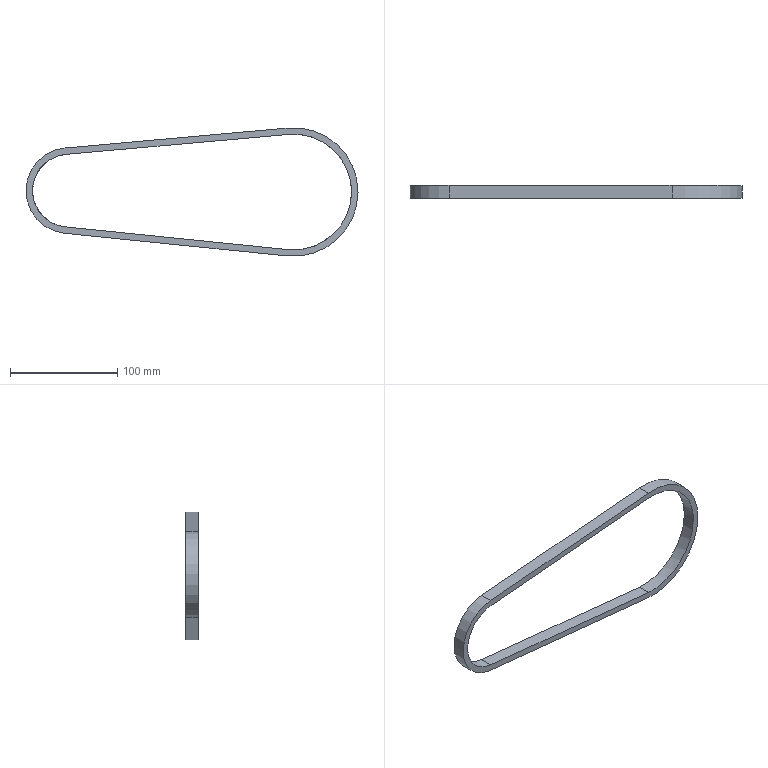Component | SolidWorks | LX-TSJ-09-1 | 1 solid | 12 faces | box 310 x 12 x 120 mm | volume 51639 mm3 | cylinder 6 | plane 6 | commonest cylinder face diameters 108 x2 120 x2 80 x1 68 x1
STEP:
#1=COLOUR_RGB('',0.7922,0.8196,0.9333);
#2=FILL_AREA_STYLE_COLOUR('',#1);
#3=FILL_AREA_STYLE('',(#2));
#4=SURFACE_STYLE_FILL_AREA(#3);
#5=SURFACE_SIDE_STYLE('',(#4));
#6=SURFACE_STYLE_USAGE(.BOTH.,#5);
#7=PRESENTATION_STYLE_ASSIGNMENT((#6));
#8=CARTESIAN_POINT('',(-5.033,-18.81,-14.193));
#9=VERTEX_POINT('',#8);
#10=CARTESIAN_POINT('',(-2.717,-18.81,-16.324));
#11=VERTEX_POINT('',#10);
#12=CARTESIAN_POINT('',(-4.843,-18.81,-16.311));
#13=DIRECTION('',(-0.,1.,0.));
#14=DIRECTION('',(-1.,0.,0.006108));
#15=AXIS2_PLACEMENT_3D('',#12,#13,#14);
#16=CIRCLE('',#15,2.126);
#17=EDGE_CURVE('',#9,#11,#16,.T.);
#18=ORIENTED_EDGE('',*,*,#17,.T.);
#19=CARTESIAN_POINT('',(-2.717,-19.282,-16.324));
#20=VERTEX_POINT('',#19);
#21=CARTESIAN_POINT('',(-2.717,-18.81,-16.324));
#22=DIRECTION('',(0.,-1.,-0.));
#23=VECTOR('',#22,39.37);
#24=LINE('',#21,#23);
#25=EDGE_CURVE('',#11,#20,#24,.T.);
#26=ORIENTED_EDGE('',*,*,#25,.T.);
#27=CARTESIAN_POINT('',(-5.033,-19.282,-14.193));
#28=VERTEX_POINT('',#27);
#29=CARTESIAN_POINT('',(-5.033,-19.282,-14.193));
#30=CARTESIAN_POINT('',(-4.885,-19.282,-14.18));
#31=CARTESIAN_POINT('',(-4.738,-19.282,-14.182));
#32=CARTESIAN_POINT('',(-4.444,-19.282,-14.218));
#33=CARTESIAN_POINT('',(-4.3,-19.282,-14.25));
#34=CARTESIAN_POINT('',(-4.02,-19.282,-14.345));
#35=CARTESIAN_POINT('',(-3.886,-19.282,-14.407));
#36=CARTESIAN_POINT('',(-3.631,-19.282,-14.558));
#37=CARTESIAN_POINT('',(-3.513,-19.282,-14.646));
#38=CARTESIAN_POINT('',(-3.295,-19.282,-14.847));
#39=CARTESIAN_POINT('',(-3.197,-19.282,-14.957));
#40=CARTESIAN_POINT('',(-3.026,-19.282,-15.199));
#41=CARTESIAN_POINT('',(-2.953,-19.282,-15.327));
#42=CARTESIAN_POINT('',(-2.835,-19.282,-15.598));
#43=CARTESIAN_POINT('',(-2.79,-19.282,-15.739));
#44=CARTESIAN_POINT('',(-2.731,-19.282,-16.029));
#45=CARTESIAN_POINT('',(-2.717,-19.282,-16.176));
#46=CARTESIAN_POINT('',(-2.717,-19.282,-16.324));
#47=B_SPLINE_CURVE_WITH_KNOTS('',3,(#29,#30,#31,#32,#33,#34,#35,#36,#37,#38,#39,#40,#41,#42,#43,#44,#45,#46),.UNSPECIFIED.,.F.,.F.,(4,2,2,2,2,2,2,2,4),(0.,0.0625,0.125,0.1875,0.25,0.3125,0.375,0.4375,0.5),.UNSPECIFIED.);
#48=EDGE_CURVE('',#28,#20,#47,.T.);
#49=ORIENTED_EDGE('',*,*,#48,.F.);
#50=CARTESIAN_POINT('',(-5.033,-18.81,-14.193));
#51=DIRECTION('',(0.,-1.,-0.));
#52=VECTOR('',#51,39.37);
#53=LINE('',#50,#52);
#54=EDGE_CURVE('',#9,#28,#53,.T.);
#55=ORIENTED_EDGE('',*,*,#54,.F.);
#56=EDGE_LOOP('',(#18,#26,#49,#55));
#57=FACE_OUTER_BOUND('',#56,.T.);
#58=CARTESIAN_POINT('',(-4.843,-18.81,-16.311));
#59=DIRECTION('',(0.,-1.,-0.));
#60=DIRECTION('',(1.,0.,-0.006108));
#61=AXIS2_PLACEMENT_3D('',#58,#59,#60);
#62=CYLINDRICAL_SURFACE('',#61,2.126);
#63=ADVANCED_FACE('',(#57),#62,.F.);
#64=CARTESIAN_POINT('',(-5.083,-18.81,-18.661));
#65=VERTEX_POINT('',#64);
#66=CARTESIAN_POINT('',(-2.481,-18.81,-16.325));
#67=VERTEX_POINT('',#66);
#68=CARTESIAN_POINT('',(-4.843,-18.81,-16.311));
#69=DIRECTION('',(0.,-1.,-0.));
#70=DIRECTION('',(1.,0.,-0.006108));
#71=AXIS2_PLACEMENT_3D('',#68,#69,#70);
#72=CIRCLE('',#71,2.362);
#73=EDGE_CURVE('',#65,#67,#72,.T.);
#74=ORIENTED_EDGE('',*,*,#73,.T.);
#75=CARTESIAN_POINT('',(-2.481,-19.282,-16.325));
#76=VERTEX_POINT('',#75);
#77=CARTESIAN_POINT('',(-2.481,-18.81,-16.325));
#78=DIRECTION('',(0.,-1.,-0.));
#79=VECTOR('',#78,39.37);
#80=LINE('',#77,#79);
#81=EDGE_CURVE('',#67,#76,#80,.T.);
#82=ORIENTED_EDGE('',*,*,#81,.T.);
#83=CARTESIAN_POINT('',(-5.083,-19.282,-18.661));
#84=VERTEX_POINT('',#83);
#85=CARTESIAN_POINT('',(-4.843,-19.282,-16.311));
#86=DIRECTION('',(-0.,1.,0.));
#87=DIRECTION('',(1.,0.,-0.006108));
#88=AXIS2_PLACEMENT_3D('',#85,#86,#87);
#89=CIRCLE('',#88,2.362);
#90=EDGE_CURVE('',#76,#84,#89,.T.);
#91=ORIENTED_EDGE('',*,*,#90,.T.);
#92=CARTESIAN_POINT('',(-5.083,-18.81,-18.661));
#93=DIRECTION('',(0.,-1.,-0.));
#94=VECTOR('',#93,39.37);
#95=LINE('',#92,#94);
#96=EDGE_CURVE('',#65,#84,#95,.T.);
#97=ORIENTED_EDGE('',*,*,#96,.F.);
#98=EDGE_LOOP('',(#74,#82,#91,#97));
#99=FACE_OUTER_BOUND('',#98,.T.);
#100=CARTESIAN_POINT('',(-4.843,-18.81,-16.311));
#101=DIRECTION('',(0.,-1.,-0.));
#102=DIRECTION('',(1.,0.,-0.006108));
#103=AXIS2_PLACEMENT_3D('',#100,#101,#102);
#104=CYLINDRICAL_SURFACE('',#103,2.362);
#105=ADVANCED_FACE('',(#99),#104,.T.);
#106=CARTESIAN_POINT('',(-13.251,-18.81,-14.692));
#107=VERTEX_POINT('',#106);
#108=CARTESIAN_POINT('',(-5.054,-18.81,-13.958));
#109=VERTEX_POINT('',#108);
#110=CARTESIAN_POINT('',(-13.251,-18.81,-14.692));
#111=DIRECTION('',(0.996,-0.,0.08916));
#112=VECTOR('',#111,39.37);
#113=LINE('',#110,#112);
#114=EDGE_CURVE('',#107,#109,#113,.T.);
#115=ORIENTED_EDGE('',*,*,#114,.T.);
#116=CARTESIAN_POINT('',(-4.843,-18.81,-16.311));
#117=DIRECTION('',(0.,-1.,-0.));
#118=DIRECTION('',(1.,0.,-0.006108));
#119=AXIS2_PLACEMENT_3D('',#116,#117,#118);
#120=CIRCLE('',#119,2.362);
#121=EDGE_CURVE('',#67,#109,#120,.T.);
#122=ORIENTED_EDGE('',*,*,#121,.F.);
#123=ORIENTED_EDGE('',*,*,#73,.F.);
#124=CARTESIAN_POINT('',(-13.271,-18.81,-17.827));
#125=VERTEX_POINT('',#124);
#126=CARTESIAN_POINT('',(-5.083,-18.81,-18.661));
#127=DIRECTION('',(-0.9949,-0.,0.1013));
#128=VECTOR('',#127,39.37);
#129=LINE('',#126,#128);
#130=EDGE_CURVE('',#65,#125,#129,.T.);
#131=ORIENTED_EDGE('',*,*,#130,.T.);
#132=CARTESIAN_POINT('',(-13.111,-18.81,-16.26));
#133=DIRECTION('',(-0.,1.,0.));
#134=DIRECTION('',(-1.,0.,0.006108));
#135=AXIS2_PLACEMENT_3D('',#132,#133,#134);
#136=CIRCLE('',#135,1.575);
#137=EDGE_CURVE('',#125,#107,#136,.T.);
#138=ORIENTED_EDGE('',*,*,#137,.T.);
#139=EDGE_LOOP('',(#115,#122,#123,#131,#138));
#140=FACE_OUTER_BOUND('',#139,.T.);
#141=CARTESIAN_POINT('',(-5.059,-18.81,-18.426));
#142=VERTEX_POINT('',#141);
#143=CARTESIAN_POINT('',(-13.247,-18.81,-17.592));
#144=VERTEX_POINT('',#143);
#145=CARTESIAN_POINT('',(-5.059,-18.81,-18.426));
#146=DIRECTION('',(-0.9949,-0.,0.1013));
#147=VECTOR('',#146,39.37);
#148=LINE('',#145,#147);
#149=EDGE_CURVE('',#142,#144,#148,.T.);
#150=ORIENTED_EDGE('',*,*,#149,.F.);
#151=CARTESIAN_POINT('',(-4.843,-18.81,-16.311));
#152=DIRECTION('',(-0.,1.,0.));
#153=DIRECTION('',(-1.,0.,0.006108));
#154=AXIS2_PLACEMENT_3D('',#151,#152,#153);
#155=CIRCLE('',#154,2.126);
#156=EDGE_CURVE('',#11,#142,#155,.T.);
#157=ORIENTED_EDGE('',*,*,#156,.F.);
#158=ORIENTED_EDGE('',*,*,#17,.F.);
#159=CARTESIAN_POINT('',(-13.23,-18.81,-14.927));
#160=VERTEX_POINT('',#159);
#161=CARTESIAN_POINT('',(-13.23,-18.81,-14.927));
#162=DIRECTION('',(0.996,-0.,0.08916));
#163=VECTOR('',#162,39.37);
#164=LINE('',#161,#163);
#165=EDGE_CURVE('',#160,#9,#164,.T.);
#166=ORIENTED_EDGE('',*,*,#165,.F.);
#167=CARTESIAN_POINT('',(-13.111,-18.81,-16.26));
#168=DIRECTION('',(-0.,1.,0.));
#169=DIRECTION('',(-1.,0.,0.006108));
#170=AXIS2_PLACEMENT_3D('',#167,#168,#169);
#171=CIRCLE('',#170,1.339);
#172=EDGE_CURVE('',#144,#160,#171,.T.);
#173=ORIENTED_EDGE('',*,*,#172,.F.);
#174=EDGE_LOOP('',(#150,#157,#158,#166,#173));
#175=FACE_BOUND('',#174,.T.);
#176=CARTESIAN_POINT('',(-4.843,-18.81,-16.311));
#177=DIRECTION('',(-0.,1.,0.));
#178=DIRECTION('',(-1.,-0.,0.006108));
#179=AXIS2_PLACEMENT_3D('',#176,#177,#178);
#180=PLANE('',#179);
#181=ADVANCED_FACE('',(#140,#175),#180,.T.);
#182=CARTESIAN_POINT('',(-13.23,-19.282,-14.927));
#183=VERTEX_POINT('',#182);
#184=CARTESIAN_POINT('',(-13.23,-19.282,-14.927));
#185=DIRECTION('',(0.996,-0.,0.08916));
#186=VECTOR('',#185,39.37);
#187=LINE('',#184,#186);
#188=EDGE_CURVE('',#183,#28,#187,.T.);
#189=ORIENTED_EDGE('',*,*,#188,.T.);
#190=ORIENTED_EDGE('',*,*,#48,.T.);
#191=CARTESIAN_POINT('',(-5.059,-19.282,-18.426));
#192=VERTEX_POINT('',#191);
#193=CARTESIAN_POINT('',(-2.717,-19.282,-16.324));
#194=CARTESIAN_POINT('',(-2.718,-19.282,-16.472));
#195=CARTESIAN_POINT('',(-2.735,-19.282,-16.619));
#196=CARTESIAN_POINT('',(-2.798,-19.282,-16.908));
#197=CARTESIAN_POINT('',(-2.844,-19.282,-17.048));
#198=CARTESIAN_POINT('',(-2.965,-19.282,-17.318));
#199=CARTESIAN_POINT('',(-3.039,-19.282,-17.445));
#200=CARTESIAN_POINT('',(-3.214,-19.282,-17.685));
#201=CARTESIAN_POINT('',(-3.313,-19.282,-17.794));
#202=CARTESIAN_POINT('',(-3.533,-19.282,-17.992));
#203=CARTESIAN_POINT('',(-3.653,-19.282,-18.078));
#204=CARTESIAN_POINT('',(-3.909,-19.282,-18.226));
#205=CARTESIAN_POINT('',(-4.044,-19.282,-18.286));
#206=CARTESIAN_POINT('',(-4.325,-19.282,-18.378));
#207=CARTESIAN_POINT('',(-4.47,-19.282,-18.409));
#208=CARTESIAN_POINT('',(-4.764,-19.282,-18.441));
#209=CARTESIAN_POINT('',(-4.911,-19.282,-18.441));
#210=CARTESIAN_POINT('',(-5.059,-19.282,-18.426));
#211=B_SPLINE_CURVE_WITH_KNOTS('',3,(#193,#194,#195,#196,#197,#198,#199,#200,#201,#202,#203,#204,#205,#206,#207,#208,#209,#210),.UNSPECIFIED.,.F.,.F.,(4,2,2,2,2,2,2,2,4),(0.5,0.5625,0.625,0.6875,0.75,0.8125,0.875,0.9375,1.),.UNSPECIFIED.);
#212=EDGE_CURVE('',#20,#192,#211,.T.);
#213=ORIENTED_EDGE('',*,*,#212,.T.);
#214=CARTESIAN_POINT('',(-13.247,-19.282,-17.592));
#215=VERTEX_POINT('',#214);
#216=CARTESIAN_POINT('',(-5.059,-19.282,-18.426));
#217=DIRECTION('',(-0.9949,-0.,0.1013));
#218=VECTOR('',#217,39.37);
#219=LINE('',#216,#218);
#220=EDGE_CURVE('',#192,#215,#219,.T.);
#221=ORIENTED_EDGE('',*,*,#220,.T.);
#222=CARTESIAN_POINT('',(-13.247,-19.282,-17.592));
#223=CARTESIAN_POINT('',(-13.329,-19.282,-17.584));
#224=CARTESIAN_POINT('',(-13.409,-19.282,-17.568));
#225=CARTESIAN_POINT('',(-13.568,-19.282,-17.521));
#226=CARTESIAN_POINT('',(-13.644,-19.282,-17.491));
#227=CARTESIAN_POINT('',(-13.791,-19.282,-17.416));
#228=CARTESIAN_POINT('',(-13.861,-19.282,-17.372));
#229=CARTESIAN_POINT('',(-13.992,-19.282,-17.272));
#230=CARTESIAN_POINT('',(-14.052,-19.282,-17.216));
#231=CARTESIAN_POINT('',(-14.162,-19.282,-17.093));
#232=CARTESIAN_POINT('',(-14.211,-19.282,-17.027));
#233=CARTESIAN_POINT('',(-14.297,-19.282,-16.886));
#234=CARTESIAN_POINT('',(-14.333,-19.282,-16.813));
#235=CARTESIAN_POINT('',(-14.392,-19.282,-16.658));
#236=CARTESIAN_POINT('',(-14.414,-19.282,-16.579));
#237=CARTESIAN_POINT('',(-14.443,-19.282,-16.417));
#238=CARTESIAN_POINT('',(-14.45,-19.282,-16.335));
#239=CARTESIAN_POINT('',(-14.449,-19.282,-16.17));
#240=CARTESIAN_POINT('',(-14.441,-19.282,-16.088));
#241=CARTESIAN_POINT('',(-14.41,-19.282,-15.926));
#242=CARTESIAN_POINT('',(-14.387,-19.282,-15.847));
#243=CARTESIAN_POINT('',(-14.326,-19.282,-15.693));
#244=CARTESIAN_POINT('',(-14.289,-19.282,-15.62));
#245=CARTESIAN_POINT('',(-14.202,-19.282,-15.48));
#246=CARTESIAN_POINT('',(-14.152,-19.282,-15.415));
#247=CARTESIAN_POINT('',(-14.04,-19.282,-15.293));
#248=CARTESIAN_POINT('',(-13.979,-19.282,-15.238));
#249=CARTESIAN_POINT('',(-13.847,-19.282,-15.139));
#250=CARTESIAN_POINT('',(-13.777,-19.282,-15.096));
#251=CARTESIAN_POINT('',(-13.629,-19.282,-15.023));
#252=CARTESIAN_POINT('',(-13.552,-19.282,-14.994));
#253=CARTESIAN_POINT('',(-13.393,-19.282,-14.949));
#254=CARTESIAN_POINT('',(-13.312,-19.282,-14.935));
#255=CARTESIAN_POINT('',(-13.23,-19.282,-14.927));
#256=B_SPLINE_CURVE_WITH_KNOTS('',3,(#222,#223,#224,#225,#226,#227,#228,#229,#230,#231,#232,#233,#234,#235,#236,#237,#238,#239,#240,#241,#242,#243,#244,#245,#246,#247,#248,#249,#250,#251,#252,#253,#254,#255),.UNSPECIFIED.,.F.,.F.,(4,2,2,2,2,2,2,2,2,2,2,2,2,2,2,2,4),(0.,0.0625,0.125,0.1875,0.25,0.3125,0.375,0.4375,0.5,0.5625,0.625,0.6875,0.75,0.8125,0.875,0.9375,1.),.UNSPECIFIED.);
#257=EDGE_CURVE('',#215,#183,#256,.T.);
#258=ORIENTED_EDGE('',*,*,#257,.T.);
#259=EDGE_LOOP('',(#189,#190,#213,#221,#258));
#260=FACE_BOUND('',#259,.T.);
#261=CARTESIAN_POINT('',(-5.054,-19.282,-13.958));
#262=VERTEX_POINT('',#261);
#263=CARTESIAN_POINT('',(-4.843,-19.282,-16.311));
#264=DIRECTION('',(-0.,1.,0.));
#265=DIRECTION('',(1.,0.,-0.006108));
#266=AXIS2_PLACEMENT_3D('',#263,#264,#265);
#267=CIRCLE('',#266,2.362);
#268=EDGE_CURVE('',#262,#76,#267,.T.);
#269=ORIENTED_EDGE('',*,*,#268,.F.);
#270=CARTESIAN_POINT('',(-13.251,-19.282,-14.692));
#271=VERTEX_POINT('',#270);
#272=CARTESIAN_POINT('',(-13.251,-19.282,-14.692));
#273=DIRECTION('',(0.996,-0.,0.08916));
#274=VECTOR('',#273,39.37);
#275=LINE('',#272,#274);
#276=EDGE_CURVE('',#271,#262,#275,.T.);
#277=ORIENTED_EDGE('',*,*,#276,.F.);
#278=CARTESIAN_POINT('',(-13.271,-19.282,-17.827));
#279=VERTEX_POINT('',#278);
#280=CARTESIAN_POINT('',(-13.111,-19.282,-16.26));
#281=DIRECTION('',(-0.,1.,0.));
#282=DIRECTION('',(-1.,0.,0.006108));
#283=AXIS2_PLACEMENT_3D('',#280,#281,#282);
#284=CIRCLE('',#283,1.575);
#285=EDGE_CURVE('',#279,#271,#284,.T.);
#286=ORIENTED_EDGE('',*,*,#285,.F.);
#287=CARTESIAN_POINT('',(-5.083,-19.282,-18.661));
#288=DIRECTION('',(-0.9949,-0.,0.1013));
#289=VECTOR('',#288,39.37);
#290=LINE('',#287,#289);
#291=EDGE_CURVE('',#84,#279,#290,.T.);
#292=ORIENTED_EDGE('',*,*,#291,.F.);
#293=ORIENTED_EDGE('',*,*,#90,.F.);
#294=EDGE_LOOP('',(#269,#277,#286,#292,#293));
#295=FACE_OUTER_BOUND('',#294,.T.);
#296=CARTESIAN_POINT('',(-4.843,-19.282,-16.311));
#297=DIRECTION('',(-0.,1.,0.));
#298=DIRECTION('',(-1.,-0.,0.006108));
#299=AXIS2_PLACEMENT_3D('',#296,#297,#298);
#300=PLANE('',#299);
#301=ADVANCED_FACE('',(#260,#295),#300,.F.);
#302=ORIENTED_EDGE('',*,*,#81,.F.);
#303=ORIENTED_EDGE('',*,*,#121,.T.);
#304=CARTESIAN_POINT('',(-5.054,-18.81,-13.958));
#305=DIRECTION('',(0.,-1.,-0.));
#306=VECTOR('',#305,39.37);
#307=LINE('',#304,#306);
#308=EDGE_CURVE('',#109,#262,#307,.T.);
#309=ORIENTED_EDGE('',*,*,#308,.T.);
#310=ORIENTED_EDGE('',*,*,#268,.T.);
#311=EDGE_LOOP('',(#302,#303,#309,#310));
#312=FACE_OUTER_BOUND('',#311,.T.);
#313=CARTESIAN_POINT('',(-4.843,-18.81,-16.311));
#314=DIRECTION('',(0.,-1.,-0.));
#315=DIRECTION('',(1.,0.,-0.006108));
#316=AXIS2_PLACEMENT_3D('',#313,#314,#315);
#317=CYLINDRICAL_SURFACE('',#316,2.362);
#318=ADVANCED_FACE('',(#312),#317,.T.);
#319=ORIENTED_EDGE('',*,*,#291,.T.);
#320=CARTESIAN_POINT('',(-13.271,-18.81,-17.827));
#321=DIRECTION('',(0.,-1.,-0.));
#322=VECTOR('',#321,39.37);
#323=LINE('',#320,#322);
#324=EDGE_CURVE('',#125,#279,#323,.T.);
#325=ORIENTED_EDGE('',*,*,#324,.F.);
#326=ORIENTED_EDGE('',*,*,#130,.F.);
#327=ORIENTED_EDGE('',*,*,#96,.T.);
#328=EDGE_LOOP('',(#319,#325,#326,#327));
#329=FACE_OUTER_BOUND('',#328,.T.);
#330=CARTESIAN_POINT('',(-5.083,-18.81,-18.661));
#331=DIRECTION('',(0.1013,-0.,0.9949));
#332=DIRECTION('',(0.9949,0.,-0.1013));
#333=AXIS2_PLACEMENT_3D('',#330,#331,#332);
#334=PLANE('',#333);
#335=ADVANCED_FACE('',(#329),#334,.F.);
#336=ORIENTED_EDGE('',*,*,#285,.T.);
#337=CARTESIAN_POINT('',(-13.251,-18.81,-14.692));
#338=DIRECTION('',(0.,-1.,-0.));
#339=VECTOR('',#338,39.37);
#340=LINE('',#337,#339);
#341=EDGE_CURVE('',#107,#271,#340,.T.);
#342=ORIENTED_EDGE('',*,*,#341,.F.);
#343=ORIENTED_EDGE('',*,*,#137,.F.);
#344=ORIENTED_EDGE('',*,*,#324,.T.);
#345=EDGE_LOOP('',(#336,#342,#343,#344));
#346=FACE_OUTER_BOUND('',#345,.T.);
#347=CARTESIAN_POINT('',(-13.111,-18.81,-16.26));
#348=DIRECTION('',(0.,-1.,-0.));
#349=DIRECTION('',(1.,0.,-0.006108));
#350=AXIS2_PLACEMENT_3D('',#347,#348,#349);
#351=CYLINDRICAL_SURFACE('',#350,1.575);
#352=ADVANCED_FACE('',(#346),#351,.T.);
#353=ORIENTED_EDGE('',*,*,#276,.T.);
#354=ORIENTED_EDGE('',*,*,#308,.F.);
#355=ORIENTED_EDGE('',*,*,#114,.F.);
#356=ORIENTED_EDGE('',*,*,#341,.T.);
#357=EDGE_LOOP('',(#353,#354,#355,#356));
#358=FACE_OUTER_BOUND('',#357,.T.);
#359=CARTESIAN_POINT('',(-13.251,-18.81,-14.692));
#360=DIRECTION('',(0.08916,0.,-0.996));
#361=DIRECTION('',(-0.996,0.,-0.08916));
#362=AXIS2_PLACEMENT_3D('',#359,#360,#361);
#363=PLANE('',#362);
#364=ADVANCED_FACE('',(#358),#363,.F.);
#365=ORIENTED_EDGE('',*,*,#25,.F.);
#366=ORIENTED_EDGE('',*,*,#156,.T.);
#367=CARTESIAN_POINT('',(-5.059,-18.81,-18.426));
#368=DIRECTION('',(0.,-1.,-0.));
#369=VECTOR('',#368,39.37);
#370=LINE('',#367,#369);
#371=EDGE_CURVE('',#142,#192,#370,.T.);
#372=ORIENTED_EDGE('',*,*,#371,.T.);
#373=ORIENTED_EDGE('',*,*,#212,.F.);
#374=EDGE_LOOP('',(#365,#366,#372,#373));
#375=FACE_OUTER_BOUND('',#374,.T.);
#376=CARTESIAN_POINT('',(-4.843,-18.81,-16.311));
#377=DIRECTION('',(0.,-1.,-0.));
#378=DIRECTION('',(1.,0.,-0.006108));
#379=AXIS2_PLACEMENT_3D('',#376,#377,#378);
#380=CYLINDRICAL_SURFACE('',#379,2.126);
#381=ADVANCED_FACE('',(#375),#380,.F.);
#382=ORIENTED_EDGE('',*,*,#220,.F.);
#383=ORIENTED_EDGE('',*,*,#371,.F.);
#384=ORIENTED_EDGE('',*,*,#149,.T.);
#385=CARTESIAN_POINT('',(-13.247,-18.81,-17.592));
#386=DIRECTION('',(0.,-1.,-0.));
#387=VECTOR('',#386,39.37);
#388=LINE('',#385,#387);
#389=EDGE_CURVE('',#144,#215,#388,.T.);
#390=ORIENTED_EDGE('',*,*,#389,.T.);
#391=EDGE_LOOP('',(#382,#383,#384,#390));
#392=FACE_OUTER_BOUND('',#391,.T.);
#393=CARTESIAN_POINT('',(-5.059,-18.81,-18.426));
#394=DIRECTION('',(0.1013,-0.,0.9949));
#395=DIRECTION('',(0.9949,0.,-0.1013));
#396=AXIS2_PLACEMENT_3D('',#393,#394,#395);
#397=PLANE('',#396);
#398=ADVANCED_FACE('',(#392),#397,.T.);
#399=ORIENTED_EDGE('',*,*,#257,.F.);
#400=ORIENTED_EDGE('',*,*,#389,.F.);
#401=ORIENTED_EDGE('',*,*,#172,.T.);
#402=CARTESIAN_POINT('',(-13.23,-18.81,-14.927));
#403=DIRECTION('',(0.,-1.,-0.));
#404=VECTOR('',#403,39.37);
#405=LINE('',#402,#404);
#406=EDGE_CURVE('',#160,#183,#405,.T.);
#407=ORIENTED_EDGE('',*,*,#406,.T.);
#408=EDGE_LOOP('',(#399,#400,#401,#407));
#409=FACE_OUTER_BOUND('',#408,.T.);
#410=CARTESIAN_POINT('',(-13.111,-18.81,-16.26));
#411=DIRECTION('',(0.,-1.,-0.));
#412=DIRECTION('',(1.,0.,-0.006108));
#413=AXIS2_PLACEMENT_3D('',#410,#411,#412);
#414=CYLINDRICAL_SURFACE('',#413,1.339);
#415=ADVANCED_FACE('',(#409),#414,.F.);
#416=ORIENTED_EDGE('',*,*,#188,.F.);
#417=ORIENTED_EDGE('',*,*,#406,.F.);
#418=ORIENTED_EDGE('',*,*,#165,.T.);
#419=ORIENTED_EDGE('',*,*,#54,.T.);
#420=EDGE_LOOP('',(#416,#417,#418,#419));
#421=FACE_OUTER_BOUND('',#420,.T.);
#422=CARTESIAN_POINT('',(-13.23,-18.81,-14.927));
#423=DIRECTION('',(0.08916,0.,-0.996));
#424=DIRECTION('',(-0.996,0.,-0.08916));
#425=AXIS2_PLACEMENT_3D('',#422,#423,#424);
#426=PLANE('',#425);
#427=ADVANCED_FACE('',(#421),#426,.T.);
#428=CLOSED_SHELL('',(#63,#105,#181,#301,#318,#335,#352,#364,#381,#398,#415,#427));
#429=MANIFOLD_SOLID_BREP('',#428);
#430=STYLED_ITEM('',(#7),#429);
#431=(LENGTH_UNIT()NAMED_UNIT(*)SI_UNIT($,.METRE.));
#432=LENGTH_MEASURE_WITH_UNIT(LENGTH_MEASURE(0.0254),#431);
#433=DIMENSIONAL_EXPONENTS(1.,0.,0.,0.,0.,0.,0.);
#434=(CONVERSION_BASED_UNIT('',#432)LENGTH_UNIT()NAMED_UNIT(#433));
#435=UNCERTAINTY_MEASURE_WITH_UNIT(LENGTH_MEASURE(0.00001),#434,'','');
#436=(NAMED_UNIT(*)PLANE_ANGLE_UNIT()SI_UNIT($,.RADIAN.));
#437=(NAMED_UNIT(*)SI_UNIT($,.STERADIAN.)SOLID_ANGLE_UNIT());
#438=(GEOMETRIC_REPRESENTATION_CONTEXT(3)GLOBAL_UNCERTAINTY_ASSIGNED_CONTEXT((#435))GLOBAL_UNIT_ASSIGNED_CONTEXT((#434,#436,#437))REPRESENTATION_CONTEXT('',''));
#439=MECHANICAL_DESIGN_GEOMETRIC_PRESENTATION_REPRESENTATION('',(#430),#438);
#440=PRESENTATION_LAYER_ASSIGNMENT('','',(#430));
#441=CARTESIAN_POINT('',(0.,0.,0.));
#442=DIRECTION('',(0.,0.,1.));
#443=DIRECTION('',(1.,0.,0.));
#444=AXIS2_PLACEMENT_3D('',#441,#442,#443);
#445=(LENGTH_UNIT()NAMED_UNIT(*)SI_UNIT($,.METRE.));
#446=LENGTH_MEASURE_WITH_UNIT(LENGTH_MEASURE(0.0254),#445);
#447=DIMENSIONAL_EXPONENTS(1.,0.,0.,0.,0.,0.,0.);
#448=(CONVERSION_BASED_UNIT('',#446)LENGTH_UNIT()NAMED_UNIT(#447));
#449=UNCERTAINTY_MEASURE_WITH_UNIT(LENGTH_MEASURE(0.00001),#448,'','');
#450=(NAMED_UNIT(*)PLANE_ANGLE_UNIT()SI_UNIT($,.RADIAN.));
#451=(NAMED_UNIT(*)SI_UNIT($,.STERADIAN.)SOLID_ANGLE_UNIT());
#452=(GEOMETRIC_REPRESENTATION_CONTEXT(3)GLOBAL_UNCERTAINTY_ASSIGNED_CONTEXT((#449))GLOBAL_UNIT_ASSIGNED_CONTEXT((#448,#450,#451))REPRESENTATION_CONTEXT('',''));
#453=ADVANCED_BREP_SHAPE_REPRESENTATION('',(#429,#444),#452);